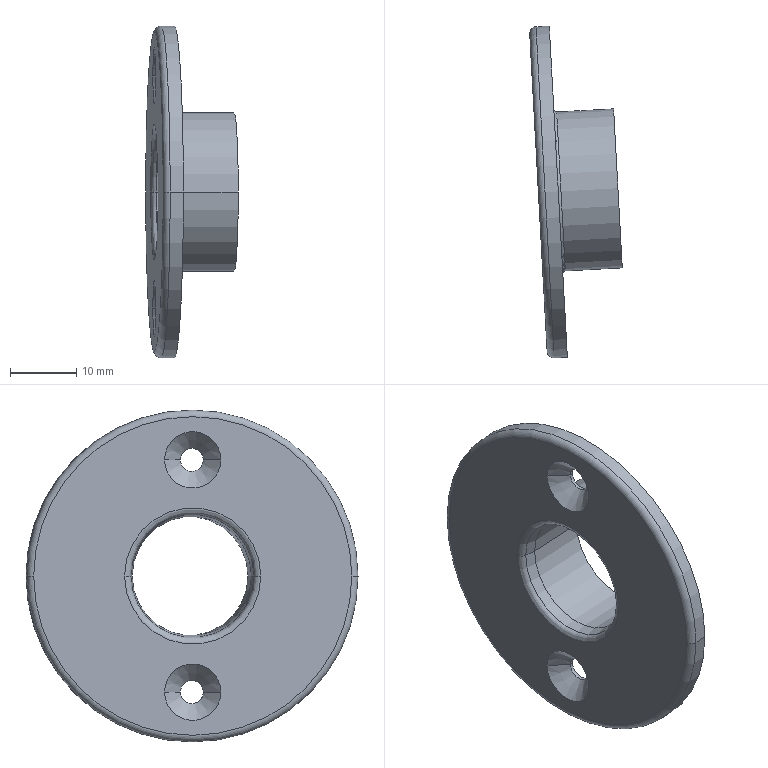Component | SolidWorks | MPSZ18-20-2 | 1 solid | 25 faces | box 13.95 x 50.04 x 50 mm | volume 6678 mm3 | cylinder 10 | cone 6 | torus 6 | plane 3 | commonest cylinder face diameters 3.5 x4 50 x2 24 x2 18 x2 | material Tin Bronze
build123d program:
from build123d import *

# Parameters (mm, degrees)
SKETCH4_W          = 57.816
SKETCH4_H          = 48.249
CUT_EXTRUDE1_DEPTH = 8


with BuildPart() as part:
    # Sketch1 → Revolve1 (revolve)
    with BuildSketch(Plane.XY, mode=Mode.PRIVATE) as revolve1_sk:
        with BuildLine():
            Line((0, 24), (0, 10.28))
            ThreePointArc((0, 10.28), (0.234, 9.637), (0.8264, 9.295))
            Line((0.8264, 9.295), (2.5, 9))
            Line((2.5, 9), (19, 9))
            ThreePointArc((19, 9), (19.707, 9.293), (20, 10))
            Line((20, 10), (20, 11.464))
            Line((20, 11.464), (18, 12))
            Line((18, 12), (3.4, 12))
            ThreePointArc((3.4, 12), (3.117, 12.117), (3, 12.4))
            Line((3, 12.4), (3, 25))
            Line((3, 25), (1, 25))
            ThreePointArc((1, 25), (0.2929, 24.707), (0, 24))
        make_face()
    revolve(revolve1_sk.sketch.rotate(Axis((20, 0, 0), (-1, 0, 0)), 270), axis=Axis((20, 0, 0), (-1, 0, 0)))

    # Sketch2 → Cut-Revolve1 (revolve, cut)
    with BuildSketch(Plane.XY, mode=Mode.PRIVATE) as cut_revolve1_sk:
        Polygon((0, 17.5), (0, 21.75), (2.5, 19.25), (3, 19.25), (3, 17.5), align=None)
    revolve(cut_revolve1_sk.sketch.rotate(Axis((3, 17.5, 0), (-1, 0, 0)), 270), axis=Axis((3, 17.5, 0), (-1, 0, 0)), mode=Mode.SUBTRACT)

    # Sketch3 → Cut-Revolve2 (revolve, cut)
    with BuildSketch(Plane.XY, mode=Mode.PRIVATE) as cut_revolve2_sk:
        Polygon((0, -17.5), (0, -13.25), (2.5, -15.75), (3, -15.75), (3, -17.5), align=None)
    revolve(cut_revolve2_sk.sketch.rotate(Axis((3, -17.5, 0), (-1, 0, 0)), 270), axis=Axis((3, -17.5, 0), (-1, 0, 0)), mode=Mode.SUBTRACT)

    # Sketch4 → Cut-Extrude1 (cut)
    with BuildSketch(Plane(origin=(20, 0, 0), x_dir=(0, 0, -1), z_dir=(1, 0, 0))):
        with Locations((-1.686, -0.6195)):
            Rectangle(SKETCH4_W, SKETCH4_H)
    extrude(amount=-CUT_EXTRUDE1_DEPTH, mode=Mode.SUBTRACT)


solid = part.part

# Placed as in the assembly
solid = solid.moved(Location((401.751, 103.414, -217.818), (-90, -3.137, 0)))
STEP:
#1=COLOUR_RGB('',0.7922,0.8196,0.9333);
#2=FILL_AREA_STYLE_COLOUR('',#1);
#3=FILL_AREA_STYLE('',(#2));
#4=SURFACE_STYLE_FILL_AREA(#3);
#5=SURFACE_SIDE_STYLE('',(#4));
#6=SURFACE_STYLE_USAGE(.BOTH.,#5);
#7=PRESENTATION_STYLE_ASSIGNMENT((#6));
#8=CARTESIAN_POINT('',(15.939,4.009,-7.887));
#9=VERTEX_POINT('',#8);
#10=CARTESIAN_POINT('',(15.931,4.147,-7.887));
#11=VERTEX_POINT('',#10);
#12=CARTESIAN_POINT('',(15.935,4.078,-7.887));
#13=DIRECTION('',(-0.9985,-0.05472,0.));
#14=DIRECTION('',(-0.05472,0.9985,0.));
#15=AXIS2_PLACEMENT_3D('',#12,#13,#14);
#16=CIRCLE('',#15,0.0689);
#17=EDGE_CURVE('',#9,#11,#16,.T.);
#18=ORIENTED_EDGE('',*,*,#17,.F.);
#19=CARTESIAN_POINT('',(15.919,4.008,-7.887));
#20=VERTEX_POINT('',#19);
#21=CARTESIAN_POINT('',(15.939,4.009,-7.887));
#22=DIRECTION('',(-0.9985,-0.05472,0.));
#23=VECTOR('',#22,39.37);
#24=LINE('',#21,#23);
#25=EDGE_CURVE('',#9,#20,#24,.T.);
#26=ORIENTED_EDGE('',*,*,#25,.T.);
#27=CARTESIAN_POINT('',(15.911,4.146,-7.887));
#28=VERTEX_POINT('',#27);
#29=CARTESIAN_POINT('',(15.915,4.077,-7.887));
#30=DIRECTION('',(-0.9985,-0.05472,0.));
#31=DIRECTION('',(-0.05472,0.9985,0.));
#32=AXIS2_PLACEMENT_3D('',#29,#30,#31);
#33=CIRCLE('',#32,0.0689);
#34=EDGE_CURVE('',#20,#28,#33,.T.);
#35=ORIENTED_EDGE('',*,*,#34,.T.);
#36=CARTESIAN_POINT('',(15.931,4.147,-7.887));
#37=DIRECTION('',(-0.9985,-0.05472,0.));
#38=VECTOR('',#37,39.37);
#39=LINE('',#36,#38);
#40=EDGE_CURVE('',#11,#28,#39,.T.);
#41=ORIENTED_EDGE('',*,*,#40,.F.);
#42=EDGE_LOOP('',(#18,#26,#35,#41));
#43=FACE_OUTER_BOUND('',#42,.T.);
#44=CARTESIAN_POINT('',(15.935,4.078,-7.887));
#45=DIRECTION('',(-0.9985,-0.05472,0.));
#46=DIRECTION('',(-0.05472,0.9985,0.));
#47=AXIS2_PLACEMENT_3D('',#44,#45,#46);
#48=CYLINDRICAL_SURFACE('',#47,0.0689);
#49=ADVANCED_FACE('',(#43),#48,.F.);
#50=ORIENTED_EDGE('',*,*,#34,.F.);
#51=CARTESIAN_POINT('',(15.826,3.904,-7.887));
#52=VERTEX_POINT('',#51);
#53=CARTESIAN_POINT('',(15.919,4.008,-7.887));
#54=DIRECTION('',(-0.6674,-0.7447,-0.));
#55=VECTOR('',#54,39.37);
#56=LINE('',#53,#55);
#57=EDGE_CURVE('',#20,#52,#56,.T.);
#58=ORIENTED_EDGE('',*,*,#57,.T.);
#59=CARTESIAN_POINT('',(15.808,4.238,-7.887));
#60=VERTEX_POINT('',#59);
#61=CARTESIAN_POINT('',(15.817,4.071,-7.887));
#62=DIRECTION('',(-0.9985,-0.05472,0.));
#63=DIRECTION('',(-0.05472,0.9985,0.));
#64=AXIS2_PLACEMENT_3D('',#61,#62,#63);
#65=CIRCLE('',#64,0.1673);
#66=EDGE_CURVE('',#52,#60,#65,.T.);
#67=ORIENTED_EDGE('',*,*,#66,.T.);
#68=CARTESIAN_POINT('',(15.911,4.146,-7.887));
#69=DIRECTION('',(-0.7447,0.6674,0.));
#70=VECTOR('',#69,39.37);
#71=LINE('',#68,#70);
#72=EDGE_CURVE('',#28,#60,#71,.T.);
#73=ORIENTED_EDGE('',*,*,#72,.F.);
#74=EDGE_LOOP('',(#50,#58,#67,#73));
#75=FACE_OUTER_BOUND('',#74,.T.);
#76=CARTESIAN_POINT('',(15.915,4.077,-7.887));
#77=DIRECTION('',(-0.9985,-0.05472,0.));
#78=DIRECTION('',(-0.05472,0.9985,0.));
#79=AXIS2_PLACEMENT_3D('',#76,#77,#78);
#80=CONICAL_SURFACE('',#79,0.0689,0.7854);
#81=ADVANCED_FACE('',(#75),#80,.F.);
#82=CARTESIAN_POINT('',(15.939,4.009,-9.264));
#83=VERTEX_POINT('',#82);
#84=CARTESIAN_POINT('',(15.931,4.147,-9.264));
#85=VERTEX_POINT('',#84);
#86=CARTESIAN_POINT('',(15.935,4.078,-9.264));
#87=DIRECTION('',(-0.9985,-0.05472,0.));
#88=DIRECTION('',(-0.05472,0.9985,0.));
#89=AXIS2_PLACEMENT_3D('',#86,#87,#88);
#90=CIRCLE('',#89,0.0689);
#91=EDGE_CURVE('',#83,#85,#90,.T.);
#92=ORIENTED_EDGE('',*,*,#91,.F.);
#93=CARTESIAN_POINT('',(15.919,4.008,-9.264));
#94=VERTEX_POINT('',#93);
#95=CARTESIAN_POINT('',(15.939,4.009,-9.264));
#96=DIRECTION('',(-0.9985,-0.05472,0.));
#97=VECTOR('',#96,39.37);
#98=LINE('',#95,#97);
#99=EDGE_CURVE('',#83,#94,#98,.T.);
#100=ORIENTED_EDGE('',*,*,#99,.T.);
#101=CARTESIAN_POINT('',(15.911,4.146,-9.264));
#102=VERTEX_POINT('',#101);
#103=CARTESIAN_POINT('',(15.915,4.077,-9.264));
#104=DIRECTION('',(-0.9985,-0.05472,0.));
#105=DIRECTION('',(-0.05472,0.9985,0.));
#106=AXIS2_PLACEMENT_3D('',#103,#104,#105);
#107=CIRCLE('',#106,0.0689);
#108=EDGE_CURVE('',#94,#102,#107,.T.);
#109=ORIENTED_EDGE('',*,*,#108,.T.);
#110=CARTESIAN_POINT('',(15.931,4.147,-9.264));
#111=DIRECTION('',(-0.9985,-0.05472,0.));
#112=VECTOR('',#111,39.37);
#113=LINE('',#110,#112);
#114=EDGE_CURVE('',#85,#102,#113,.T.);
#115=ORIENTED_EDGE('',*,*,#114,.F.);
#116=EDGE_LOOP('',(#92,#100,#109,#115));
#117=FACE_OUTER_BOUND('',#116,.T.);
#118=CARTESIAN_POINT('',(15.935,4.078,-9.264));
#119=DIRECTION('',(-0.9985,-0.05472,0.));
#120=DIRECTION('',(-0.05472,0.9985,0.));
#121=AXIS2_PLACEMENT_3D('',#118,#119,#120);
#122=CYLINDRICAL_SURFACE('',#121,0.0689);
#123=ADVANCED_FACE('',(#117),#122,.F.);
#124=ORIENTED_EDGE('',*,*,#108,.F.);
#125=CARTESIAN_POINT('',(15.826,3.904,-9.264));
#126=VERTEX_POINT('',#125);
#127=CARTESIAN_POINT('',(15.919,4.008,-9.264));
#128=DIRECTION('',(-0.6674,-0.7447,-0.));
#129=VECTOR('',#128,39.37);
#130=LINE('',#127,#129);
#131=EDGE_CURVE('',#94,#126,#130,.T.);
#132=ORIENTED_EDGE('',*,*,#131,.T.);
#133=CARTESIAN_POINT('',(15.808,4.238,-9.264));
#134=VERTEX_POINT('',#133);
#135=CARTESIAN_POINT('',(15.817,4.071,-9.264));
#136=DIRECTION('',(-0.9985,-0.05472,0.));
#137=DIRECTION('',(-0.05472,0.9985,0.));
#138=AXIS2_PLACEMENT_3D('',#135,#136,#137);
#139=CIRCLE('',#138,0.1673);
#140=EDGE_CURVE('',#126,#134,#139,.T.);
#141=ORIENTED_EDGE('',*,*,#140,.T.);
#142=CARTESIAN_POINT('',(15.911,4.146,-9.264));
#143=DIRECTION('',(-0.7447,0.6674,0.));
#144=VECTOR('',#143,39.37);
#145=LINE('',#142,#144);
#146=EDGE_CURVE('',#102,#134,#145,.T.);
#147=ORIENTED_EDGE('',*,*,#146,.F.);
#148=EDGE_LOOP('',(#124,#132,#141,#147));
#149=FACE_OUTER_BOUND('',#148,.T.);
#150=CARTESIAN_POINT('',(15.915,4.077,-9.264));
#151=DIRECTION('',(-0.9985,-0.05472,0.));
#152=DIRECTION('',(-0.05472,0.9985,0.));
#153=AXIS2_PLACEMENT_3D('',#150,#151,#152);
#154=CONICAL_SURFACE('',#153,0.0689,0.7854);
#155=ADVANCED_FACE('',(#149),#154,.F.);
#156=CARTESIAN_POINT('',(15.881,5.061,-8.576));
#157=VERTEX_POINT('',#156);
#158=CARTESIAN_POINT('',(15.989,3.095,-8.576));
#159=VERTEX_POINT('',#158);
#160=CARTESIAN_POINT('',(15.935,4.078,-8.576));
#161=DIRECTION('',(-0.9985,-0.05472,0.));
#162=DIRECTION('',(-0.05472,0.9985,0.));
#163=AXIS2_PLACEMENT_3D('',#160,#161,#162);
#164=CIRCLE('',#163,0.9843);
#165=EDGE_CURVE('',#157,#159,#164,.T.);
#166=ORIENTED_EDGE('',*,*,#165,.T.);
#167=CARTESIAN_POINT('',(15.91,3.091,-8.576));
#168=VERTEX_POINT('',#167);
#169=CARTESIAN_POINT('',(16.657,3.132,-8.576));
#170=DIRECTION('',(-0.9985,-0.05472,0.));
#171=VECTOR('',#170,39.37);
#172=LINE('',#169,#171);
#173=EDGE_CURVE('',#159,#168,#172,.T.);
#174=ORIENTED_EDGE('',*,*,#173,.T.);
#175=CARTESIAN_POINT('',(15.802,5.056,-8.576));
#176=VERTEX_POINT('',#175);
#177=CARTESIAN_POINT('',(15.856,4.074,-8.576));
#178=DIRECTION('',(-0.9985,-0.05472,0.));
#179=DIRECTION('',(-0.05472,0.9985,0.));
#180=AXIS2_PLACEMENT_3D('',#177,#178,#179);
#181=CIRCLE('',#180,0.9843);
#182=EDGE_CURVE('',#176,#168,#181,.T.);
#183=ORIENTED_EDGE('',*,*,#182,.F.);
#184=CARTESIAN_POINT('',(16.549,5.097,-8.576));
#185=DIRECTION('',(-0.9985,-0.05472,0.));
#186=VECTOR('',#185,39.37);
#187=LINE('',#184,#186);
#188=EDGE_CURVE('',#157,#176,#187,.T.);
#189=ORIENTED_EDGE('',*,*,#188,.F.);
#190=EDGE_LOOP('',(#166,#174,#183,#189));
#191=FACE_OUTER_BOUND('',#190,.T.);
#192=CARTESIAN_POINT('',(16.603,4.115,-8.576));
#193=DIRECTION('',(-0.9985,-0.05472,0.));
#194=DIRECTION('',(-0.05472,0.9985,0.));
#195=AXIS2_PLACEMENT_3D('',#192,#193,#194);
#196=CYLINDRICAL_SURFACE('',#195,0.9843);
#197=ADVANCED_FACE('',(#191),#196,.T.);
#198=CARTESIAN_POINT('',(15.962,3.59,-8.576));
#199=VERTEX_POINT('',#198);
#200=CARTESIAN_POINT('',(15.908,4.565,-8.576));
#201=VERTEX_POINT('',#200);
#202=CARTESIAN_POINT('',(15.935,4.078,-8.576));
#203=DIRECTION('',(-0.9985,-0.05472,0.));
#204=DIRECTION('',(-0.05472,0.9985,0.));
#205=AXIS2_PLACEMENT_3D('',#202,#203,#204);
#206=CIRCLE('',#205,0.4882);
#207=EDGE_CURVE('',#199,#201,#206,.T.);
#208=ORIENTED_EDGE('',*,*,#207,.F.);
#209=CARTESIAN_POINT('',(15.976,3.607,-8.576));
#210=VERTEX_POINT('',#209);
#211=CARTESIAN_POINT('',(15.977,3.591,-8.576));
#212=DIRECTION('',(-0.,0.,-1.));
#213=DIRECTION('',(0.,1.,0.));
#214=AXIS2_PLACEMENT_3D('',#211,#212,#213);
#215=CIRCLE('',#214,0.01575);
#216=EDGE_CURVE('',#199,#210,#215,.T.);
#217=ORIENTED_EDGE('',*,*,#216,.T.);
#218=CARTESIAN_POINT('',(15.925,4.55,-8.576));
#219=VERTEX_POINT('',#218);
#220=CARTESIAN_POINT('',(15.951,4.079,-8.576));
#221=DIRECTION('',(-0.9985,-0.05472,0.));
#222=DIRECTION('',(-0.05472,0.9985,0.));
#223=AXIS2_PLACEMENT_3D('',#220,#221,#222);
#224=CIRCLE('',#223,0.4724);
#225=EDGE_CURVE('',#210,#219,#224,.T.);
#226=ORIENTED_EDGE('',*,*,#225,.T.);
#227=CARTESIAN_POINT('',(15.924,4.566,-8.576));
#228=DIRECTION('',(0.,-0.,1.));
#229=DIRECTION('',(0.,-1.,0.));
#230=AXIS2_PLACEMENT_3D('',#227,#228,#229);
#231=CIRCLE('',#230,0.01575);
#232=EDGE_CURVE('',#201,#219,#231,.T.);
#233=ORIENTED_EDGE('',*,*,#232,.F.);
#234=EDGE_LOOP('',(#208,#217,#226,#233));
#235=FACE_OUTER_BOUND('',#234,.T.);
#236=CARTESIAN_POINT('',(15.951,4.079,-8.576));
#237=DIRECTION('',(-0.9985,-0.05472,0.));
#238=DIRECTION('',(-0.05472,0.9985,-0.));
#239=AXIS2_PLACEMENT_3D('',#236,#237,#238);
#240=TOROIDAL_SURFACE('',#239,0.4882,0.01575);
#241=ADVANCED_FACE('',(#235),#240,.F.);
#242=CARTESIAN_POINT('',(15.935,3.723,-8.576));
#243=VERTEX_POINT('',#242);
#244=CARTESIAN_POINT('',(15.896,4.431,-8.576));
#245=VERTEX_POINT('',#244);
#246=CARTESIAN_POINT('',(15.915,4.077,-8.576));
#247=DIRECTION('',(-0.9985,-0.05472,0.));
#248=DIRECTION('',(-0.05472,0.9985,0.));
#249=AXIS2_PLACEMENT_3D('',#246,#247,#248);
#250=CIRCLE('',#249,0.3543);
#251=EDGE_CURVE('',#243,#245,#250,.T.);
#252=ORIENTED_EDGE('',*,*,#251,.F.);
#253=CARTESIAN_POINT('',(15.869,3.708,-8.576));
#254=VERTEX_POINT('',#253);
#255=CARTESIAN_POINT('',(15.869,3.708,-8.576));
#256=DIRECTION('',(-0.9738,-0.2273,0.));
#257=VECTOR('',#256,39.37);
#258=LINE('',#255,#257);
#259=EDGE_CURVE('',#243,#254,#258,.T.);
#260=ORIENTED_EDGE('',*,*,#259,.T.);
#261=CARTESIAN_POINT('',(15.829,4.439,-8.576));
#262=VERTEX_POINT('',#261);
#263=CARTESIAN_POINT('',(15.849,4.073,-8.576));
#264=DIRECTION('',(-0.9985,-0.05472,0.));
#265=DIRECTION('',(-0.05472,0.9985,0.));
#266=AXIS2_PLACEMENT_3D('',#263,#264,#265);
#267=CIRCLE('',#266,0.3659);
#268=EDGE_CURVE('',#254,#262,#267,.T.);
#269=ORIENTED_EDGE('',*,*,#268,.T.);
#270=CARTESIAN_POINT('',(15.829,4.439,-8.576));
#271=DIRECTION('',(-0.9928,0.1195,0.));
#272=VECTOR('',#271,39.37);
#273=LINE('',#270,#272);
#274=EDGE_CURVE('',#245,#262,#273,.T.);
#275=ORIENTED_EDGE('',*,*,#274,.F.);
#276=EDGE_LOOP('',(#252,#260,#269,#275));
#277=FACE_OUTER_BOUND('',#276,.T.);
#278=CARTESIAN_POINT('',(15.849,4.073,-8.576));
#279=DIRECTION('',(-0.9985,-0.05472,0.));
#280=DIRECTION('',(-0.05472,0.9985,0.));
#281=AXIS2_PLACEMENT_3D('',#278,#279,#280);
#282=CONICAL_SURFACE('',#281,0.3659,0.1745);
#283=ADVANCED_FACE('',(#277),#282,.F.);
#284=CARTESIAN_POINT('',(15.795,4.476,-8.576));
#285=VERTEX_POINT('',#284);
#286=CARTESIAN_POINT('',(15.839,3.667,-8.576));
#287=VERTEX_POINT('',#286);
#288=CARTESIAN_POINT('',(15.817,4.071,-8.576));
#289=DIRECTION('',(-0.9985,-0.05472,0.));
#290=DIRECTION('',(-0.05472,0.9985,0.));
#291=AXIS2_PLACEMENT_3D('',#288,#289,#290);
#292=CIRCLE('',#291,0.4047);
#293=EDGE_CURVE('',#285,#287,#292,.T.);
#294=ORIENTED_EDGE('',*,*,#293,.T.);
#295=CARTESIAN_POINT('',(15.878,3.669,-8.576));
#296=DIRECTION('',(-0.,0.,-1.));
#297=DIRECTION('',(0.,1.,0.));
#298=AXIS2_PLACEMENT_3D('',#295,#296,#297);
#299=CIRCLE('',#298,0.03937);
#300=EDGE_CURVE('',#287,#254,#299,.T.);
#301=ORIENTED_EDGE('',*,*,#300,.T.);
#302=CARTESIAN_POINT('',(15.849,4.073,-8.576));
#303=DIRECTION('',(-0.9985,-0.05472,0.));
#304=DIRECTION('',(-0.05472,0.9985,0.));
#305=AXIS2_PLACEMENT_3D('',#302,#303,#304);
#306=CIRCLE('',#305,0.3659);
#307=EDGE_CURVE('',#262,#254,#306,.T.);
#308=ORIENTED_EDGE('',*,*,#307,.F.);
#309=CARTESIAN_POINT('',(15.834,4.478,-8.576));
#310=DIRECTION('',(0.,-0.,1.));
#311=DIRECTION('',(0.,-1.,0.));
#312=AXIS2_PLACEMENT_3D('',#309,#310,#311);
#313=CIRCLE('',#312,0.03937);
#314=EDGE_CURVE('',#285,#262,#313,.T.);
#315=ORIENTED_EDGE('',*,*,#314,.F.);
#316=EDGE_LOOP('',(#294,#301,#308,#315));
#317=FACE_OUTER_BOUND('',#316,.T.);
#318=CARTESIAN_POINT('',(15.856,4.074,-8.576));
#319=DIRECTION('',(-0.9985,-0.05472,0.));
#320=DIRECTION('',(-0.05472,0.9985,0.));
#321=AXIS2_PLACEMENT_3D('',#318,#319,#320);
#322=TOROIDAL_SURFACE('',#321,0.4047,0.03937);
#323=ADVANCED_FACE('',(#317),#322,.T.);
#324=ORIENTED_EDGE('',*,*,#182,.T.);
#325=CARTESIAN_POINT('',(15.869,3.128,-8.576));
#326=VERTEX_POINT('',#325);
#327=CARTESIAN_POINT('',(15.908,3.13,-8.576));
#328=DIRECTION('',(-0.,0.,-1.));
#329=DIRECTION('',(0.,1.,0.));
#330=AXIS2_PLACEMENT_3D('',#327,#328,#329);
#331=CIRCLE('',#330,0.03937);
#332=EDGE_CURVE('',#168,#326,#331,.T.);
#333=ORIENTED_EDGE('',*,*,#332,.T.);
#334=CARTESIAN_POINT('',(15.765,5.015,-8.576));
#335=VERTEX_POINT('',#334);
#336=CARTESIAN_POINT('',(15.817,4.071,-8.576));
#337=DIRECTION('',(-0.9985,-0.05472,0.));
#338=DIRECTION('',(-0.05472,0.9985,0.));
#339=AXIS2_PLACEMENT_3D('',#336,#337,#338);
#340=CIRCLE('',#339,0.9449);
#341=EDGE_CURVE('',#335,#326,#340,.T.);
#342=ORIENTED_EDGE('',*,*,#341,.F.);
#343=CARTESIAN_POINT('',(15.805,5.017,-8.576));
#344=DIRECTION('',(0.,-0.,1.));
#345=DIRECTION('',(0.,-1.,0.));
#346=AXIS2_PLACEMENT_3D('',#343,#344,#345);
#347=CIRCLE('',#346,0.03937);
#348=EDGE_CURVE('',#176,#335,#347,.T.);
#349=ORIENTED_EDGE('',*,*,#348,.F.);
#350=EDGE_LOOP('',(#324,#333,#342,#349));
#351=FACE_OUTER_BOUND('',#350,.T.);
#352=CARTESIAN_POINT('',(15.856,4.074,-8.576));
#353=DIRECTION('',(-0.9985,-0.05472,0.));
#354=DIRECTION('',(-0.05472,0.9985,-0.));
#355=AXIS2_PLACEMENT_3D('',#352,#353,#354);
#356=TOROIDAL_SURFACE('',#355,0.9449,0.03937);
#357=ADVANCED_FACE('',(#351),#356,.T.);
#358=CARTESIAN_POINT('',(16.315,3.626,-8.576));
#359=VERTEX_POINT('',#358);
#360=CARTESIAN_POINT('',(16.263,4.569,-8.576));
#361=VERTEX_POINT('',#360);
#362=CARTESIAN_POINT('',(16.289,4.097,-8.576));
#363=DIRECTION('',(0.9985,0.05472,-0.));
#364=DIRECTION('',(0.05472,-0.9985,0.));
#365=AXIS2_PLACEMENT_3D('',#362,#363,#364);
#366=CIRCLE('',#365,0.4724);
#367=EDGE_CURVE('',#359,#361,#366,.T.);
#368=ORIENTED_EDGE('',*,*,#367,.F.);
#369=CARTESIAN_POINT('',(16.629,3.643,-8.576));
#370=DIRECTION('',(-0.9985,-0.05472,0.));
#371=VECTOR('',#370,39.37);
#372=LINE('',#369,#371);
#373=EDGE_CURVE('',#359,#210,#372,.T.);
#374=ORIENTED_EDGE('',*,*,#373,.T.);
#375=CARTESIAN_POINT('',(15.951,4.079,-8.576));
#376=DIRECTION('',(-0.9985,-0.05472,0.));
#377=DIRECTION('',(-0.05472,0.9985,0.));
#378=AXIS2_PLACEMENT_3D('',#375,#376,#377);
#379=CIRCLE('',#378,0.4724);
#380=EDGE_CURVE('',#219,#210,#379,.T.);
#381=ORIENTED_EDGE('',*,*,#380,.F.);
#382=CARTESIAN_POINT('',(16.577,4.586,-8.576));
#383=DIRECTION('',(-0.9985,-0.05472,0.));
#384=VECTOR('',#383,39.37);
#385=LINE('',#382,#384);
#386=EDGE_CURVE('',#361,#219,#385,.T.);
#387=ORIENTED_EDGE('',*,*,#386,.F.);
#388=EDGE_LOOP('',(#368,#374,#381,#387));
#389=FACE_OUTER_BOUND('',#388,.T.);
#390=CARTESIAN_POINT('',(16.603,4.115,-8.576));
#391=DIRECTION('',(-0.9985,-0.05472,0.));
#392=DIRECTION('',(-0.05472,0.9985,0.));
#393=AXIS2_PLACEMENT_3D('',#390,#391,#392);
#394=CYLINDRICAL_SURFACE('',#393,0.4724);
#395=ADVANCED_FACE('',(#389),#394,.T.);
#396=CARTESIAN_POINT('',(16.308,3.743,-8.576));
#397=VERTEX_POINT('',#396);
#398=CARTESIAN_POINT('',(16.269,4.451,-8.576));
#399=VERTEX_POINT('',#398);
#400=CARTESIAN_POINT('',(16.289,4.097,-8.576));
#401=DIRECTION('',(-0.9985,-0.05472,0.));
#402=DIRECTION('',(0.05472,-0.9985,0.));
#403=AXIS2_PLACEMENT_3D('',#400,#401,#402);
#404=CIRCLE('',#403,0.3543);
#405=EDGE_CURVE('',#397,#399,#404,.T.);
#406=ORIENTED_EDGE('',*,*,#405,.F.);
#407=CARTESIAN_POINT('',(16.623,3.761,-8.576));
#408=DIRECTION('',(-0.9985,-0.05472,0.));
#409=VECTOR('',#408,39.37);
#410=LINE('',#407,#409);
#411=EDGE_CURVE('',#397,#243,#410,.T.);
#412=ORIENTED_EDGE('',*,*,#411,.T.);
#413=ORIENTED_EDGE('',*,*,#251,.T.);
#414=CARTESIAN_POINT('',(16.584,4.468,-8.576));
#415=DIRECTION('',(-0.9985,-0.05472,0.));
#416=VECTOR('',#415,39.37);
#417=LINE('',#414,#416);
#418=EDGE_CURVE('',#399,#245,#417,.T.);
#419=ORIENTED_EDGE('',*,*,#418,.F.);
#420=EDGE_LOOP('',(#406,#412,#413,#419));
#421=FACE_OUTER_BOUND('',#420,.T.);
#422=CARTESIAN_POINT('',(16.603,4.115,-8.576));
#423=DIRECTION('',(-0.9985,-0.05472,0.));
#424=DIRECTION('',(-0.05472,0.9985,0.));
#425=AXIS2_PLACEMENT_3D('',#422,#423,#424);
#426=CYLINDRICAL_SURFACE('',#425,0.3543);
#427=ADVANCED_FACE('',(#421),#426,.F.);
#428=ORIENTED_EDGE('',*,*,#411,.F.);
#429=CARTESIAN_POINT('',(16.289,4.097,-8.576));
#430=DIRECTION('',(-0.9985,-0.05472,0.));
#431=DIRECTION('',(0.05472,-0.9985,0.));
#432=AXIS2_PLACEMENT_3D('',#429,#430,#431);
#433=CIRCLE('',#432,0.3543);
#434=EDGE_CURVE('',#399,#397,#433,.T.);
#435=ORIENTED_EDGE('',*,*,#434,.F.);
#436=ORIENTED_EDGE('',*,*,#418,.T.);
#437=CARTESIAN_POINT('',(15.915,4.077,-8.576));
#438=DIRECTION('',(-0.9985,-0.05472,0.));
#439=DIRECTION('',(-0.05472,0.9985,0.));
#440=AXIS2_PLACEMENT_3D('',#437,#438,#439);
#441=CIRCLE('',#440,0.3543);
#442=EDGE_CURVE('',#245,#243,#441,.T.);
#443=ORIENTED_EDGE('',*,*,#442,.T.);
#444=EDGE_LOOP('',(#428,#435,#436,#443));
#445=FACE_OUTER_BOUND('',#444,.T.);
#446=CARTESIAN_POINT('',(16.603,4.115,-8.576));
#447=DIRECTION('',(-0.9985,-0.05472,0.));
#448=DIRECTION('',(-0.05472,0.9985,0.));
#449=AXIS2_PLACEMENT_3D('',#446,#447,#448);
#450=CYLINDRICAL_SURFACE('',#449,0.3543);
#451=ADVANCED_FACE('',(#445),#450,.F.);
#452=ORIENTED_EDGE('',*,*,#373,.F.);
#453=CARTESIAN_POINT('',(16.289,4.097,-8.576));
#454=DIRECTION('',(0.9985,0.05472,-0.));
#455=DIRECTION('',(0.05472,-0.9985,0.));
#456=AXIS2_PLACEMENT_3D('',#453,#454,#455);
#457=CIRCLE('',#456,0.4724);
#458=EDGE_CURVE('',#361,#359,#457,.T.);
#459=ORIENTED_EDGE('',*,*,#458,.F.);
#460=ORIENTED_EDGE('',*,*,#386,.T.);
#461=ORIENTED_EDGE('',*,*,#225,.F.);
#462=EDGE_LOOP('',(#452,#459,#460,#461));
#463=FACE_OUTER_BOUND('',#462,.T.);
#464=CARTESIAN_POINT('',(16.603,4.115,-8.576));
#465=DIRECTION('',(-0.9985,-0.05472,0.));
#466=DIRECTION('',(-0.05472,0.9985,0.));
#467=AXIS2_PLACEMENT_3D('',#464,#465,#466);
#468=CYLINDRICAL_SURFACE('',#467,0.4724);
#469=ADVANCED_FACE('',(#463),#468,.T.);
#470=ORIENTED_EDGE('',*,*,#293,.F.);
#471=CARTESIAN_POINT('',(15.817,4.071,-8.576));
#472=DIRECTION('',(-0.9985,-0.05472,0.));
#473=DIRECTION('',(-0.05472,0.9985,0.));
#474=AXIS2_PLACEMENT_3D('',#471,#472,#473);
#475=CIRCLE('',#474,0.4047);
#476=EDGE_CURVE('',#287,#285,#475,.T.);
#477=ORIENTED_EDGE('',*,*,#476,.F.);
#478=EDGE_LOOP('',(#470,#477));
#479=FACE_BOUND('',#478,.T.);
#480=ORIENTED_EDGE('',*,*,#341,.T.);
#481=CARTESIAN_POINT('',(15.817,4.071,-8.576));
#482=DIRECTION('',(-0.9985,-0.05472,0.));
#483=DIRECTION('',(-0.05472,0.9985,0.));
#484=AXIS2_PLACEMENT_3D('',#481,#482,#483);
#485=CIRCLE('',#484,0.9449);
#486=EDGE_CURVE('',#326,#335,#485,.T.);
#487=ORIENTED_EDGE('',*,*,#486,.T.);
#488=EDGE_LOOP('',(#480,#487));
#489=FACE_OUTER_BOUND('',#488,.T.);
#490=CARTESIAN_POINT('',(15.817,4.071,-9.264));
#491=DIRECTION('',(-0.9985,-0.05472,0.));
#492=DIRECTION('',(-0.05472,0.9985,0.));
#493=AXIS2_PLACEMENT_3D('',#490,#491,#492);
#494=CIRCLE('',#493,0.1673);
#495=EDGE_CURVE('',#134,#126,#494,.T.);
#496=ORIENTED_EDGE('',*,*,#495,.F.);
#497=ORIENTED_EDGE('',*,*,#140,.F.);
#498=EDGE_LOOP('',(#496,#497));
#499=FACE_BOUND('',#498,.T.);
#500=CARTESIAN_POINT('',(15.817,4.071,-7.887));
#501=DIRECTION('',(-0.9985,-0.05472,0.));
#502=DIRECTION('',(-0.05472,0.9985,0.));
#503=AXIS2_PLACEMENT_3D('',#500,#501,#502);
#504=CIRCLE('',#503,0.1673);
#505=EDGE_CURVE('',#60,#52,#504,.T.);
#506=ORIENTED_EDGE('',*,*,#505,.F.);
#507=ORIENTED_EDGE('',*,*,#66,.F.);
#508=EDGE_LOOP('',(#506,#507));
#509=FACE_BOUND('',#508,.T.);
#510=CARTESIAN_POINT('',(15.817,4.071,-9.52));
#511=DIRECTION('',(0.9985,0.05472,-0.));
#512=DIRECTION('',(0.05472,-0.9985,-0.));
#513=AXIS2_PLACEMENT_3D('',#510,#511,#512);
#514=PLANE('',#513);
#515=ADVANCED_FACE('',(#479,#489,#499,#509),#514,.F.);
#516=ORIENTED_EDGE('',*,*,#165,.F.);
#517=CARTESIAN_POINT('',(15.935,4.078,-8.576));
#518=DIRECTION('',(-0.9985,-0.05472,0.));
#519=DIRECTION('',(-0.05472,0.9985,0.));
#520=AXIS2_PLACEMENT_3D('',#517,#518,#519);
#521=CIRCLE('',#520,0.9843);
#522=EDGE_CURVE('',#159,#157,#521,.T.);
#523=ORIENTED_EDGE('',*,*,#522,.F.);
#524=EDGE_LOOP('',(#516,#523));
#525=FACE_OUTER_BOUND('',#524,.T.);
#526=CARTESIAN_POINT('',(15.935,4.078,-8.576));
#527=DIRECTION('',(-0.9985,-0.05472,0.));
#528=DIRECTION('',(-0.05472,0.9985,0.));
#529=AXIS2_PLACEMENT_3D('',#526,#527,#528);
#530=CIRCLE('',#529,0.4882);
#531=EDGE_CURVE('',#201,#199,#530,.T.);
#532=ORIENTED_EDGE('',*,*,#531,.T.);
#533=ORIENTED_EDGE('',*,*,#207,.T.);
#534=EDGE_LOOP('',(#532,#533));
#535=FACE_BOUND('',#534,.T.);
#536=CARTESIAN_POINT('',(15.935,4.078,-9.264));
#537=DIRECTION('',(-0.9985,-0.05472,0.));
#538=DIRECTION('',(-0.05472,0.9985,0.));
#539=AXIS2_PLACEMENT_3D('',#536,#537,#538);
#540=CIRCLE('',#539,0.0689);
#541=EDGE_CURVE('',#85,#83,#540,.T.);
#542=ORIENTED_EDGE('',*,*,#541,.T.);
#543=ORIENTED_EDGE('',*,*,#91,.T.);
#544=EDGE_LOOP('',(#542,#543));
#545=FACE_BOUND('',#544,.T.);
#546=CARTESIAN_POINT('',(15.935,4.078,-7.887));
#547=DIRECTION('',(-0.9985,-0.05472,0.));
#548=DIRECTION('',(-0.05472,0.9985,0.));
#549=AXIS2_PLACEMENT_3D('',#546,#547,#548);
#550=CIRCLE('',#549,0.0689);
#551=EDGE_CURVE('',#11,#9,#550,.T.);
#552=ORIENTED_EDGE('',*,*,#551,.T.);
#553=ORIENTED_EDGE('',*,*,#17,.T.);
#554=EDGE_LOOP('',(#552,#553));
#555=FACE_BOUND('',#554,.T.);
#556=CARTESIAN_POINT('',(15.935,4.078,-9.064));
#557=DIRECTION('',(-0.9985,-0.05472,0.));
#558=DIRECTION('',(-0.05472,0.9985,0.));
#559=AXIS2_PLACEMENT_3D('',#556,#557,#558);
#560=PLANE('',#559);
#561=ADVANCED_FACE('',(#525,#535,#545,#555),#560,.F.);
#562=ORIENTED_EDGE('',*,*,#332,.F.);
#563=CARTESIAN_POINT('',(15.856,4.074,-8.576));
#564=DIRECTION('',(-0.9985,-0.05472,0.));
#565=DIRECTION('',(-0.05472,0.9985,0.));
#566=AXIS2_PLACEMENT_3D('',#563,#564,#565);
#567=CIRCLE('',#566,0.9843);
#568=EDGE_CURVE('',#168,#176,#567,.T.);
#569=ORIENTED_EDGE('',*,*,#568,.T.);
#570=ORIENTED_EDGE('',*,*,#348,.T.);
#571=ORIENTED_EDGE('',*,*,#486,.F.);
#572=EDGE_LOOP('',(#562,#569,#570,#571));
#573=FACE_OUTER_BOUND('',#572,.T.);
#574=CARTESIAN_POINT('',(15.856,4.074,-8.576));
#575=DIRECTION('',(-0.9985,-0.05472,0.));
#576=DIRECTION('',(-0.05472,0.9985,-0.));
#577=AXIS2_PLACEMENT_3D('',#574,#575,#576);
#578=TOROIDAL_SURFACE('',#577,0.9449,0.03937);
#579=ADVANCED_FACE('',(#573),#578,.T.);
#580=ORIENTED_EDGE('',*,*,#300,.F.);
#581=ORIENTED_EDGE('',*,*,#476,.T.);
#582=ORIENTED_EDGE('',*,*,#314,.T.);
#583=ORIENTED_EDGE('',*,*,#268,.F.);
#584=EDGE_LOOP('',(#580,#581,#582,#583));
#585=FACE_OUTER_BOUND('',#584,.T.);
#586=CARTESIAN_POINT('',(15.856,4.074,-8.576));
#587=DIRECTION('',(-0.9985,-0.05472,0.));
#588=DIRECTION('',(-0.05472,0.9985,0.));
#589=AXIS2_PLACEMENT_3D('',#586,#587,#588);
#590=TOROIDAL_SURFACE('',#589,0.4047,0.03937);
#591=ADVANCED_FACE('',(#585),#590,.T.);
#592=ORIENTED_EDGE('',*,*,#259,.F.);
#593=ORIENTED_EDGE('',*,*,#442,.F.);
#594=ORIENTED_EDGE('',*,*,#274,.T.);
#595=ORIENTED_EDGE('',*,*,#307,.T.);
#596=EDGE_LOOP('',(#592,#593,#594,#595));
#597=FACE_OUTER_BOUND('',#596,.T.);
#598=CARTESIAN_POINT('',(15.849,4.073,-8.576));
#599=DIRECTION('',(-0.9985,-0.05472,0.));
#600=DIRECTION('',(-0.05472,0.9985,0.));
#601=AXIS2_PLACEMENT_3D('',#598,#599,#600);
#602=CONICAL_SURFACE('',#601,0.3659,0.1745);
#603=ADVANCED_FACE('',(#597),#602,.F.);
#604=ORIENTED_EDGE('',*,*,#216,.F.);
#605=ORIENTED_EDGE('',*,*,#531,.F.);
#606=ORIENTED_EDGE('',*,*,#232,.T.);
#607=ORIENTED_EDGE('',*,*,#380,.T.);
#608=EDGE_LOOP('',(#604,#605,#606,#607));
#609=FACE_OUTER_BOUND('',#608,.T.);
#610=CARTESIAN_POINT('',(15.951,4.079,-8.576));
#611=DIRECTION('',(-0.9985,-0.05472,0.));
#612=DIRECTION('',(-0.05472,0.9985,-0.));
#613=AXIS2_PLACEMENT_3D('',#610,#611,#612);
#614=TOROIDAL_SURFACE('',#613,0.4882,0.01575);
#615=ADVANCED_FACE('',(#609),#614,.F.);
#616=ORIENTED_EDGE('',*,*,#173,.F.);
#617=ORIENTED_EDGE('',*,*,#522,.T.);
#618=ORIENTED_EDGE('',*,*,#188,.T.);
#619=ORIENTED_EDGE('',*,*,#568,.F.);
#620=EDGE_LOOP('',(#616,#617,#618,#619));
#621=FACE_OUTER_BOUND('',#620,.T.);
#622=CARTESIAN_POINT('',(16.603,4.115,-8.576));
#623=DIRECTION('',(-0.9985,-0.05472,0.));
#624=DIRECTION('',(-0.05472,0.9985,0.));
#625=AXIS2_PLACEMENT_3D('',#622,#623,#624);
#626=CYLINDRICAL_SURFACE('',#625,0.9843);
#627=ADVANCED_FACE('',(#621),#626,.T.);
#628=ORIENTED_EDGE('',*,*,#131,.F.);
#629=CARTESIAN_POINT('',(15.915,4.077,-9.264));
#630=DIRECTION('',(-0.9985,-0.05472,0.));
#631=DIRECTION('',(-0.05472,0.9985,0.));
#632=AXIS2_PLACEMENT_3D('',#629,#630,#631);
#633=CIRCLE('',#632,0.0689);
#634=EDGE_CURVE('',#102,#94,#633,.T.);
#635=ORIENTED_EDGE('',*,*,#634,.F.);
#636=ORIENTED_EDGE('',*,*,#146,.T.);
#637=ORIENTED_EDGE('',*,*,#495,.T.);
#638=EDGE_LOOP('',(#628,#635,#636,#637));
#639=FACE_OUTER_BOUND('',#638,.T.);
#640=CARTESIAN_POINT('',(15.915,4.077,-9.264));
#641=DIRECTION('',(-0.9985,-0.05472,0.));
#642=DIRECTION('',(-0.05472,0.9985,0.));
#643=AXIS2_PLACEMENT_3D('',#640,#641,#642);
#644=CONICAL_SURFACE('',#643,0.0689,0.7854);
#645=ADVANCED_FACE('',(#639),#644,.F.);
#646=ORIENTED_EDGE('',*,*,#99,.F.);
#647=ORIENTED_EDGE('',*,*,#541,.F.);
#648=ORIENTED_EDGE('',*,*,#114,.T.);
#649=ORIENTED_EDGE('',*,*,#634,.T.);
#650=EDGE_LOOP('',(#646,#647,#648,#649));
#651=FACE_OUTER_BOUND('',#650,.T.);
#652=CARTESIAN_POINT('',(15.935,4.078,-9.264));
#653=DIRECTION('',(-0.9985,-0.05472,0.));
#654=DIRECTION('',(-0.05472,0.9985,0.));
#655=AXIS2_PLACEMENT_3D('',#652,#653,#654);
#656=CYLINDRICAL_SURFACE('',#655,0.0689);
#657=ADVANCED_FACE('',(#651),#656,.F.);
#658=ORIENTED_EDGE('',*,*,#57,.F.);
#659=CARTESIAN_POINT('',(15.915,4.077,-7.887));
#660=DIRECTION('',(-0.9985,-0.05472,0.));
#661=DIRECTION('',(-0.05472,0.9985,0.));
#662=AXIS2_PLACEMENT_3D('',#659,#660,#661);
#663=CIRCLE('',#662,0.0689);
#664=EDGE_CURVE('',#28,#20,#663,.T.);
#665=ORIENTED_EDGE('',*,*,#664,.F.);
#666=ORIENTED_EDGE('',*,*,#72,.T.);
#667=ORIENTED_EDGE('',*,*,#505,.T.);
#668=EDGE_LOOP('',(#658,#665,#666,#667));
#669=FACE_OUTER_BOUND('',#668,.T.);
#670=CARTESIAN_POINT('',(15.915,4.077,-7.887));
#671=DIRECTION('',(-0.9985,-0.05472,0.));
#672=DIRECTION('',(-0.05472,0.9985,0.));
#673=AXIS2_PLACEMENT_3D('',#670,#671,#672);
#674=CONICAL_SURFACE('',#673,0.0689,0.7854);
#675=ADVANCED_FACE('',(#669),#674,.F.);
#676=ORIENTED_EDGE('',*,*,#25,.F.);
#677=ORIENTED_EDGE('',*,*,#551,.F.);
#678=ORIENTED_EDGE('',*,*,#40,.T.);
#679=ORIENTED_EDGE('',*,*,#664,.T.);
#680=EDGE_LOOP('',(#676,#677,#678,#679));
#681=FACE_OUTER_BOUND('',#680,.T.);
#682=CARTESIAN_POINT('',(15.935,4.078,-7.887));
#683=DIRECTION('',(-0.9985,-0.05472,0.));
#684=DIRECTION('',(-0.05472,0.9985,0.));
#685=AXIS2_PLACEMENT_3D('',#682,#683,#684);
#686=CYLINDRICAL_SURFACE('',#685,0.0689);
#687=ADVANCED_FACE('',(#681),#686,.F.);
#688=ORIENTED_EDGE('',*,*,#458,.T.);
#689=ORIENTED_EDGE('',*,*,#367,.T.);
#690=EDGE_LOOP('',(#688,#689));
#691=FACE_OUTER_BOUND('',#690,.T.);
#692=ORIENTED_EDGE('',*,*,#434,.T.);
#693=ORIENTED_EDGE('',*,*,#405,.T.);
#694=EDGE_LOOP('',(#692,#693));
#695=FACE_BOUND('',#694,.T.);
#696=CARTESIAN_POINT('',(16.289,4.097,-8.576));
#697=DIRECTION('',(0.9985,0.05472,-0.));
#698=DIRECTION('',(0.05472,-0.9985,-0.));
#699=AXIS2_PLACEMENT_3D('',#696,#697,#698);
#700=PLANE('',#699);
#701=ADVANCED_FACE('',(#691,#695),#700,.T.);
#702=CLOSED_SHELL('',(#49,#81,#123,#155,#197,#241,#283,#323,#357,#395,#427,#451,#469,#515,#561,#579,#591,#603,#615,#627,#645,#657,#675,#687,#701));
#703=MANIFOLD_SOLID_BREP('',#702);
#704=STYLED_ITEM('',(#7),#703);
#705=PRESENTATION_LAYER_ASSIGNMENT('','',(#704));
#706=CARTESIAN_POINT('',(0.,0.,0.));
#707=DIRECTION('',(0.,0.,1.));
#708=DIRECTION('',(1.,0.,0.));
#709=AXIS2_PLACEMENT_3D('',#706,#707,#708);
#710=(LENGTH_UNIT()NAMED_UNIT(*)SI_UNIT($,.METRE.));
#711=LENGTH_MEASURE_WITH_UNIT(LENGTH_MEASURE(0.0254),#710);
#712=DIMENSIONAL_EXPONENTS(1.,0.,0.,0.,0.,0.,0.);
#713=(CONVERSION_BASED_UNIT('',#711)LENGTH_UNIT()NAMED_UNIT(#712));
#714=UNCERTAINTY_MEASURE_WITH_UNIT(LENGTH_MEASURE(0.00001),#713,'','');
#715=(NAMED_UNIT(*)PLANE_ANGLE_UNIT()SI_UNIT($,.RADIAN.));
#716=(NAMED_UNIT(*)SI_UNIT($,.STERADIAN.)SOLID_ANGLE_UNIT());
#717=(GEOMETRIC_REPRESENTATION_CONTEXT(3)GLOBAL_UNCERTAINTY_ASSIGNED_CONTEXT((#714))GLOBAL_UNIT_ASSIGNED_CONTEXT((#713,#715,#716))REPRESENTATION_CONTEXT('',''));
#718=ADVANCED_BREP_SHAPE_REPRESENTATION('',(#703,#709),#717);
#719=(LENGTH_UNIT()NAMED_UNIT(*)SI_UNIT($,.METRE.));
#720=LENGTH_MEASURE_WITH_UNIT(LENGTH_MEASURE(0.0254),#719);
#721=DIMENSIONAL_EXPONENTS(1.,0.,0.,0.,0.,0.,0.);
#722=(CONVERSION_BASED_UNIT('',#720)LENGTH_UNIT()NAMED_UNIT(#721));
#723=UNCERTAINTY_MEASURE_WITH_UNIT(LENGTH_MEASURE(0.00001),#722,'','');
#724=(NAMED_UNIT(*)PLANE_ANGLE_UNIT()SI_UNIT($,.RADIAN.));
#725=(NAMED_UNIT(*)SI_UNIT($,.STERADIAN.)SOLID_ANGLE_UNIT());
#726=(GEOMETRIC_REPRESENTATION_CONTEXT(3)GLOBAL_UNCERTAINTY_ASSIGNED_CONTEXT((#723))GLOBAL_UNIT_ASSIGNED_CONTEXT((#722,#724,#725))REPRESENTATION_CONTEXT('',''));
#727=MECHANICAL_DESIGN_GEOMETRIC_PRESENTATION_REPRESENTATION('',(#704),#726);